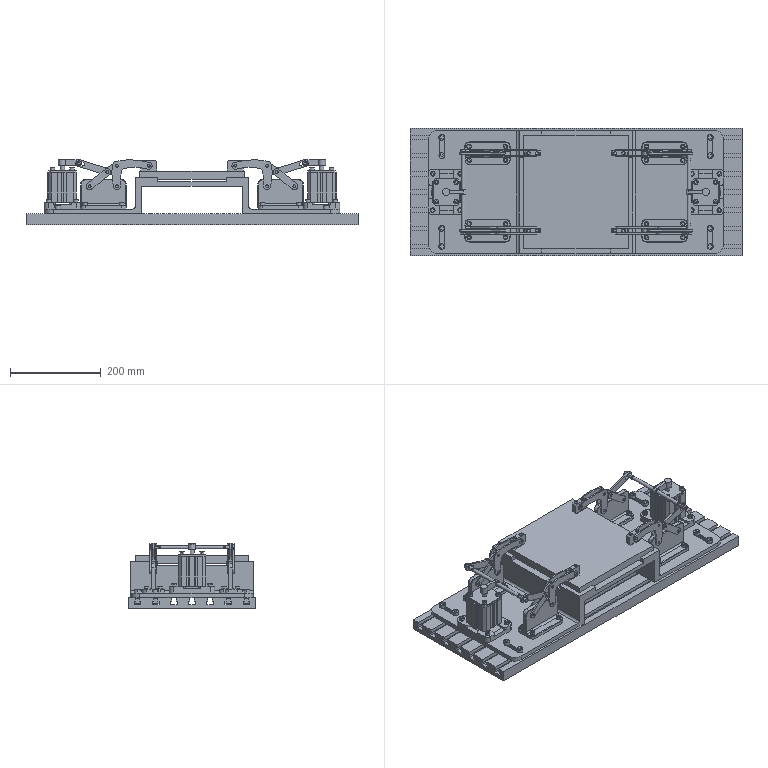Assembly | NX | mm | 119 component files | 119 solids | 2190 faces | box 730 x 280 x 144.8 mm | volume 8410763 mm3 | plane 1128 | cylinder 614 | cone 272 | torus 176 | commonest cylinder face diameters 6 x196 10 x108 8 x100 20 x68 15 x32 240 x16 13 x16 5 x16
Bill of materials:
unnamed part 1 | 8 |  | Prismatic block with a T-shaped cross-section: a narrower raised upper section on a wider base, with one vertical round through-hole in the upper face.
unnamed part 2 | 2 |  | Straight plain cylindrical rod standing up from the center of a thin circular disc base, like a flanged pin or post.
unnamed part 3 | 4 |  | Bracket with a T-shaped profile: a vertical plate with two round holes stands centered on a horizontal base flange that has four round holes, two on each side of the upright.
unnamed part 4 | 4 |  | Rectangular block with all four corners of the large face chamfered. One round through-hole goes through the large face, and two parallel round through-holes cross at right angles to it through the narrow top face.
unnamed part 5 | 2 |  | Flat square plate with chamfered corners, a larger central round through-hole, and four smaller round through-holes near the corners.
unnamed part 6 | 8 |  | Cap-screw-like solid: a cylindrical head with a hexagonal socket recess on top, a plain cylindrical shank, and a chamfered tip.
unnamed part 7 | 4 |  | Flat annular ring with rectangular cross-section, split by one narrow radial gap, like a split ring or split washer.
unnamed part 8 | 2 |  | Rectangular open frame with rounded outer corners. Four thicker raised corner pads, each with a larger and a smaller round through-hole, are joined by thinner straight bars around a large central opening.
unnamed part 9 | 8 |  | Cap-screw-like solid with a cylindrical head, a hexagonal socket recess, and a plain cylindrical shank with a chamfered tip. It is shorter and stockier than unnamed part 6.
unnamed part 10 | 1 |  | Plain thin square plate with no holes or edge features.
unnamed part 11 | 4 |  | Flat dogleg link plate: two straight arms meet at an obtuse angle in the plate's plane, with rounded ends. A long slot is at the end of the longer arm, and two round holes are on the shorter arm.
unnamed part 12 | 20 |  | Plain solid cylinder with flat ends, like a rod or pin blank.
unnamed part 13 | 2 |  | Crank-like lever: a solid cylindrical boss at one end joined by a straight, slightly tapered rectangular arm to a smaller cylindrical eye with a through bore at the other end; the eye axis is perpendicular to the boss axis.
unnamed part 14 | 1 |  | Rectangular plate of constant thickness with rounded corners, formed into a hat-shaped profile: a raised flat central section between two lower flanges. Each flange has elongated slots near its corners and a pattern of small round holes. Small notched tabs stand up at the ends of the raised section.
unnamed part 15 | 8 |  | Flat, obround link plate of uniform thickness with one round through hole near each rounded end.
unnamed part 16 | 28 |  | Cap-screw-shaped part: a cylindrical head with a hexagonal socket recess on top, over a smaller-diameter plain cylindrical shank with a chamfered end.
unnamed part 17 | 2 |  | Prismatic square-profile body with chamfered corners and a large central round through bore. Four corner holes run lengthwise. Shallow grooves and notches run the full length of the side faces, and one side has a protruding rib.
unnamed part 18 | 1 |  | Flat rectangular plate whose top face has seven parallel T-shaped slots running its full length.
unnamed part 19 | 2 |  | Long, straight, thin-walled circular tube with a constant diameter and square-cut ends.
unnamed part 20 | 8 |  | Flat L-shaped or boomerang-shaped plate of uniform thickness. Its two arms are slightly curved and meet at a filleted inside corner, with rounded ends. There are three round through holes: one at the corner and one at the end of each arm.
Mates:
1. fix | Machine_Tool_Platform 1 component
2. touch align | Machine_Tool_Platform 1 face | Machining_Platform 1 face
3. center | Machining_Platform 1 face | Machining_Platform 1 face | Machine_Tool_Platform 1 face | Machine_Tool_Platform 1 face
4. center | Machining_Platform 1 face | Machining_Platform 1 face | Machine_Tool_Platform 1 face | Machine_Tool_Platform 1 face
5. parallel | Fixed_Block 8 face | Machine_Tool_Platform 1 face
6. touch align | Fixed_Block 8 face | Machining_Platform 1 face
7. touch align | Fixed_Block 8 face | Machine_Tool_Platform 1 face
8. touch align | Fixed_Block 7 face | Machining_Platform 1 face
9. parallel | Fixed_Block 7 face | Machine_Tool_Platform 1 face
10. touch align | Fixed_Block 7 face | Machine_Tool_Platform 1 face
11. touch align | Fixed_Block 6 face | Machining_Platform 1 face
12. parallel | Fixed_Block 6 face | Machine_Tool_Platform 1 face
13. touch align | Fixed_Block 6 face | Machine_Tool_Platform 1 face
14. touch align | Fixed_Block 5 face | Machining_Platform 1 face
15. parallel | Fixed_Block 5 face | Machine_Tool_Platform 1 face
16. touch align | Fixed_Block 5 face | Machine_Tool_Platform 1 face
17. concentric | Cylinder_Base 2 arc | Machining_Platform 1 edge
18. parallel | Cylinder_Base 2 face | Machining_Platform 1 face
19. concentric | Cylinder 2 edge | Cylinder_Base 2 edge
20. parallel | Cylinder 2 face | Cylinder_Base 2 face
21. concentric | Cylinder_Base 1 arc | Machining_Platform 1 edge
22. parallel | Cylinder_Base 1 face | Machining_Platform 1 face
23. concentric | Cylinder 1 edge | Cylinder_Base 1 edge
24. parallel | Cylinder 1 face | Cylinder_Base 1 face
25. concentric | Machining_Platform 1 edge | Bracket 4 edge
26. parallel | Bracket 4 face | Machining_Platform 1 face
27. concentric | Bracket 3 edge | Machining_Platform 1 edge
28. parallel | Bracket 3 face | Machining_Platform 1 face
29. concentric | Bracket 2 edge | Machining_Platform 1 edge
30. parallel | Bracket 2 face | Machine_Tool_Platform 1 face
31. concentric | Machining_Platform 1 edge | Bracket 1 edge
32. parallel | Bracket 1 face | Machining_Platform 1 face
33. touch align | Piston 2 face | Cylinder 2 face
34. touch align | Piston 1 face | Cylinder 1 face
35. concentric | Cylinder_Cover 2 edge | Cylinder 2 edge
36. parallel | Cylinder_Cover 2 face | Cylinder 2 face
37. concentric | Cylinder 1 edge | Cylinder_Cover 1 edge
38. parallel | Cylinder_Cover 1 face | Cylinder 1 face
39. concentric | Link_2 8 edge | Bracket 2 edge
40. concentric | Link_2 7 arc | Bracket 2 edge
41. concentric | Link_2 6 arc | Bracket 1 edge
42. concentric | Link_2 5 edge | Bracket 1 edge
43. concentric | Link_2 4 arc | Bracket 3 edge
44. concentric | Link_2 3 edge | Bracket 3 edge
45. concentric | Link_2 2 arc | Bracket 4 edge
46. concentric | Link_2 1 edge | Bracket 4 edge
47. concentric | Clamping_Block 4 arc | Link_2 5 edge
48. concentric | Clamping_Block 3 arc | Link_2 2 edge
49. concentric | Clamping_Block 2 arc | Link_2 8 edge
50. concentric | Clamping_Block 1 arc | Link_2 4 edge
51. touch align | Link_3 4 face | Link_2 8 face
52. center | Link_3 4 face | Link_3 4 face | Link_2 8 face | Link_2 7 face
53. concentric | Link_1 8 arc | Bracket 2 edge
54. touch align | Link_1 8 face | Link_3 4 face
55. concentric | Link_1 7 edge | Bracket 2 edge
56. touch align | Link_1 7 face | Link_3 4 face
57. touch align | Link_3 3 face | Link_2 5 face
58. center | Link_3 3 face | Link_3 3 face | Link_2 5 face | Link_2 6 face
59. touch align | Link_2 7 face | Link_3 4 face
60. touch align | Link_3 3 face | Link_1 6 face
61. touch align | Link_2 6 face | Link_2 5 face
62. concentric | Link_1 6 arc | Bracket 1 edge
63. concentric | Link_1 5 edge | Bracket 1 edge
64. touch align | Link_1 5 face | Link_3 3 face
65. parallel | Link_3 4 face | Link_3 3 face
66. center | Connecting_Rod_2 2 face | Connecting_Rod_2 2 face | Link_3 3 face | Link_3 4 face
67. touch align | Connecting_Rod_2 2 face | Link_3 4 face
68. touch align | Link_3 2 face | Link_2 2 face
69. center | Link_3 2 face | Link_3 2 face | Link_2 2 face | Link_2 1 face
70. touch align | Link_3 1 face | Link_2 4 face
71. center | Link_3 1 face | Link_3 1 face | Link_2 4 face | Link_2 3 face
72. concentric | Link_1 4 arc | Bracket 3 edge
73. touch align | Link_1 4 face | Link_3 1 face
74. concentric | Link_1 3 edge | Bracket 3 edge
75. touch align | Link_1 3 face | Link_3 1 face
76. concentric | Link_1 2 edge | Bracket 4 edge
77. touch align | Link_3 2 face | Link_1 2 face
78. concentric | Link_1 1 arc | Bracket 4 edge
79. touch align | Link_1 1 face | Link_3 2 face
80. parallel | Link_3 2 face | Link_3 1 face
81. concentric | Link_2 1 edge | Clamping_Block 3 edge
82. concentric | Link_2 3 edge | Clamping_Block 1 edge
83. concentric | Connecting_Rod_2 1 edge | Link_3 1 arc
84. center | Connecting_Rod_1 1 face | Connecting_Rod_1 1 face | Bracket 3 face | Bracket 4 face
85. touch align | Connecting_Rod_1 1 face | Connecting_Rod_1 2 face
86. touch align | Piston 2 face | Connecting_Rod_1 1 face
87. touch align | Piston 1 face | Connecting_Rod_1 2 face
88. touch align | Connecting_Rod_1 2 face | Connecting_Rod_2 2 face
89. touch align | Connecting_Rod_1 1 face | Connecting_Rod_2 1 face
90. touch align | Machining_Platform 1 face | Workpiece 1 face
91. center | Workpiece 1 face | Workpiece 1 face | Machining_Platform 1 face | Machining_Platform 1 face
92. center | Workpiece 1 face | Workpiece 1 face | Machining_Platform 1 face | Machining_Platform 1 face
93. parallel | Clamping_Block 2 face | Workpiece 1 face
94. parallel | Clamping_Block 4 face | Workpiece 1 face
95. parallel | Clamping_Block 3 face | Workpiece 1 face
96. parallel | Clamping_Block 1 face | Workpiece 1 face
97. concentric | Connecting_Shaft 20 edge | Link_2 5 edge
98. concentric | Connecting_Shaft 19 edge | Link_2 5 edge
99. concentric | Connecting_Shaft 18 edge | Link_1 6 edge
100. concentric | Connecting_Shaft 17 edge | Link_2 5 edge
101. concentric | Connecting_Shaft 16 | Link_2 8 edge
102. concentric | Connecting_Shaft 15 edge | Link_2 8 edge
103. concentric | Connecting_Shaft 14 edge | Link_2 8 edge
104. concentric | Connecting_Shaft 13 | Link_1 8 edge
105. concentric | Connecting_Shaft 12 | Link_1 8 edge
106. concentric | Connecting_Shaft 11 edge | Link_1 6 edge
107. concentric | Connecting_Shaft 10 edge | Link_2 4 edge
108. concentric | Connecting_Shaft 9 edge | Link_2 4 edge
109. concentric | Connecting_Shaft 8 edge | Link_2 4 edge
110. concentric | Connecting_Shaft 7 edge | Link_1 4 edge
111. concentric | Connecting_Shaft 6 edge | Link_1 4 edge
112. concentric | Connecting_Shaft 5 edge | Link_2 2 edge
113. concentric | Connecting_Shaft 4 edge | Link_2 2 edge
114. concentric | Connecting_Shaft 3 edge | Link_1 1 edge
115. concentric | Connecting_Shaft 2 edge | Link_2 2 edge
116. concentric | Connecting_Shaft 1 edge | Link_1 1 edge
117. touch align | Fixed_Block 4 face | Machining_Platform 1 face
118. touch align | Fixed_Block 4 face | Machine_Tool_Platform 1 face
119. parallel | Fixed_Block 4 face | Machine_Tool_Platform 1 face
120. touch align | Fixed_Block 3 face | Machining_Platform 1 face
121. touch align | Fixed_Block 3 face | Machine_Tool_Platform 1 face
122. parallel | Fixed_Block 3 face | Machine_Tool_Platform 1 face
123. touch align | Fixed_Block 2 face | Machining_Platform 1 face
124. touch align | Fixed_Block 2 face | Machine_Tool_Platform 1 face
125. parallel | Fixed_Block 2 face | Machine_Tool_Platform 1 face
126. touch align | Fixed_Block 1 face | Machining_Platform 1 face
127. touch align | Fixed_Block 1 face | Machine_Tool_Platform 1 face
128. parallel | Fixed_Block 1 face | Machine_Tool_Platform 1 face
129. concentric | Socket_Head_Screw_M6x16 28 edge | Bracket 4 edge
130. concentric | Socket_Head_Screw_M6x16 27 edge | Bracket 4 edge
131. concentric | Socket_Head_Screw_M6x16 26 edge | Bracket 4 edge
132. concentric | Socket_Head_Screw_M6x16 25 edge | Bracket 4 edge
133. concentric | Socket_Head_Screw_M6x16 24 edge | Bracket 3 edge
134. concentric | Socket_Head_Screw_M6x16 23 edge | Bracket 3 edge
135. concentric | Socket_Head_Screw_M6x16 22 edge | Bracket 3 edge
136. concentric | Socket_Head_Screw_M6x16 21 edge | Bracket 3 edge
137. concentric | Socket_Head_Screw_M6x16 20 edge | Bracket 1 edge
138. concentric | Socket_Head_Screw_M6x16 19 edge | Bracket 1 edge
139. concentric | Socket_Head_Screw_M6x16 18 edge | Bracket 1 edge
140. concentric | Socket_Head_Screw_M6x16 17 edge | Bracket 1 edge
141. concentric | Socket_Head_Screw_M6x16 16 edge | Bracket 2 edge
142. concentric | Socket_Head_Screw_M6x16 15 edge | Bracket 2 edge
143. concentric | Socket_Head_Screw_M6x16 14 edge | Bracket 2 edge
144. concentric | Socket_Head_Screw_M6x16 13 edge | Bracket 2 edge
145. concentric | Socket_Head_Screw_M6x16 12 edge | Cylinder_Cover 1 edge
146. concentric | Socket_Head_Screw_M6x16 11 edge | Cylinder_Cover 1 edge
147. concentric | Socket_Head_Screw_M6x16 10 edge | Cylinder_Cover 1 edge
148. concentric | Socket_Head_Screw_M6x16 9 edge | Cylinder_Cover 1 edge
149. concentric | Socket_Head_Screw_M6x16 8 edge | Cylinder_Cover 2 edge
150. concentric | Socket_Head_Screw_M6x16 7 edge | Cylinder_Cover 2 edge
151. concentric | Socket_Head_Screw_M6x16 6 edge | Cylinder_Cover 2 edge
152. concentric | Socket_Head_Screw_M6x16 5 edge | Cylinder_Cover 2 edge
153. concentric | Socket_Head_Screw_M6x25 8 edge | Cylinder_Base 2 edge
154. concentric | Socket_Head_Screw_M6x25 7 edge | Cylinder_Base 2 edge
155. concentric | Socket_Head_Screw_M6x25 6 edge | Cylinder_Base 2 edge
156. concentric | Socket_Head_Screw_M6x25 5 edge | Cylinder_Base 2 edge
157. concentric | Socket_Head_Screw_M6x25 4 edge | Cylinder_Base 1 edge
158. concentric | Socket_Head_Screw_M6x25 3 | Cylinder_Base 1 edge
159. concentric | Socket_Head_Screw_M6x25 2 edge | Cylinder_Base 1 edge
160. concentric | Socket_Head_Screw_M6x25 1 edge | Cylinder_Base 1 edge
161. concentric | Socket_Head_Screw_M8x25 8 edge | Machining_Platform 1 edge
162. concentric | Socket_Head_Screw_M8x25 7 edge | Machining_Platform 1 edge
163. concentric | Socket_Head_Screw_M8x25 6 edge | Machining_Platform 1 edge
164. concentric | Socket_Head_Screw_M8x25 5 edge | Machining_Platform 1 edge
165. concentric | Socket_Head_Screw_M8x25 4 edge | Machining_Platform 1 edge
166. concentric | Socket_Head_Screw_M8x25 3 edge | Machining_Platform 1 edge
167. concentric | Socket_Head_Screw_M8x25 2 edge | Machining_Platform 1 edge
168. concentric | Socket_Head_Screw_M8x25 1 edge | Machining_Platform 1 edge
169. concentric | Wave_Spring_Washer_6 4 edge | Link_3 3 edge
170. concentric | Wave_Spring_Washer_6 3 edge | Link_3 4 edge
171. concentric | Wave_Spring_Washer_6 2 edge | Connecting_Rod_2 1 edge
172. concentric | Wave_Spring_Washer_6 1 edge | Connecting_Rod_2 1 edge
173. concentric | Socket_Head_Screw_M6x16 4 edge | Wave_Spring_Washer_6 4 edge
174. concentric | Socket_Head_Screw_M6x16 3 | Wave_Spring_Washer_6 3 edge
175. concentric | Socket_Head_Screw_M6x16 2 edge | Wave_Spring_Washer_6 2 edge
176. concentric | Socket_Head_Screw_M6x16 1 edge | Wave_Spring_Washer_6 1 edge